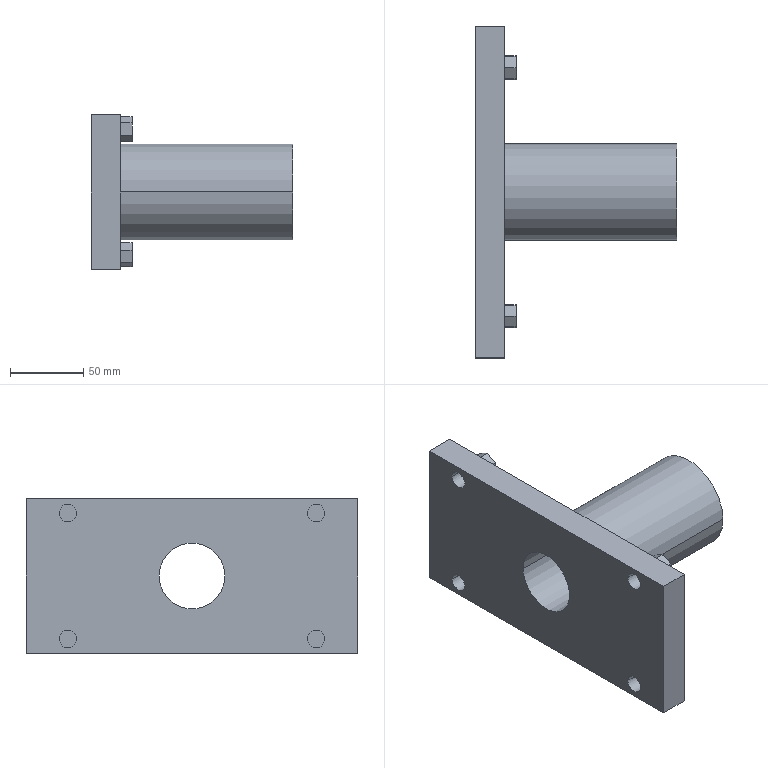Component | SolidWorks | SupportPlate3-1 | 1 solid | 51 faces | box 138 x 227 x 106 mm | volume 662407 mm3 | plane 39 | cylinder 12 | commonest cylinder face diameters 12 x8 45 x2 66 x2
build123d program:
from build123d import *

# Parameters (mm, degrees)
SKETCH1_R           = 33
SKETCH1_R_2         = 22.5
BOSS_EXTRUDE1_DEPTH = 118
SKETCH2_W           = 227
SKETCH2_H           = 106
BOSS_EXTRUDE2_DEPTH = 20
SKETCH4_R           = 22.5
CUT_EXTRUDE1_DEPTH  = 187.374
SKETCH5_R           = 6
CUT_EXTRUDE2_DEPTH  = 20
BOSS_EXTRUDE3_DEPTH = 8


with BuildPart() as part:
    # Sketch1 → Boss-Extrude1 (new body)
    with BuildSketch(Plane(origin=(0, 0, 0), x_dir=(0, 0, -1), z_dir=(1, 0, 0))):
        Circle(SKETCH1_R)
        Circle(SKETCH1_R_2, mode=Mode.SUBTRACT)
    extrude(amount=BOSS_EXTRUDE1_DEPTH)

    # Sketch2 → Boss-Extrude2 (add)
    with BuildSketch(Plane(origin=(118, 0, 0), x_dir=(0, 0, -1), z_dir=(1, 0, 0))):
        Rectangle(SKETCH2_W, SKETCH2_H)
    extrude(amount=BOSS_EXTRUDE2_DEPTH)

    # Sketch4 → Cut-Extrude1 (cut, through all)
    with BuildSketch(Plane.ZY):
        Circle(SKETCH4_R)
    extrude(amount=-CUT_EXTRUDE1_DEPTH, mode=Mode.SUBTRACT)

    # Sketch5 → Cut-Extrude2 (cut)
    with BuildSketch(Plane(origin=(138, 0, 0), x_dir=(0, 0, -1), z_dir=(1, 0, 0))):
        with Locations((-85, 43)):
            Circle(SKETCH5_R)
        with Locations((85, 43)):
            Circle(SKETCH5_R)
        with Locations((-85, -43)):
            Circle(SKETCH5_R)
        with Locations((85, -43)):
            Circle(SKETCH5_R)
    extrude(amount=-CUT_EXTRUDE2_DEPTH, mode=Mode.SUBTRACT)

    # Sketch6 → Boss-Extrude3 (add)
    with BuildSketch(Plane.ZY.offset(-118)):
        Polygon((-91, 37), (-82.804, 34.804), (-76.804, 40.804), (-79, 49), (-87.196, 51.196), (-93.196, 45.196), align=None)
        Polygon((78.484, 37.804), (86.242, 34.759), (92.758, 39.955), (91.516, 48.196), (83.758, 51.241), (77.242, 46.045), align=None)
        Polygon((-85, -51.57), (-77.578, -47.285), (-77.578, -38.715), (-85, -34.43), (-92.422, -38.715), (-92.422, -47.285), align=None)
        Polygon((85, -51.57), (92.422, -47.285), (92.422, -38.715), (85, -34.43), (77.578, -38.715), (77.578, -47.285), align=None)
    extrude(amount=BOSS_EXTRUDE3_DEPTH)


solid = part.part

# Placed as in the assembly
solid = solid.moved(Location((577.733, 15.31, -110), (90, 0, -180)))